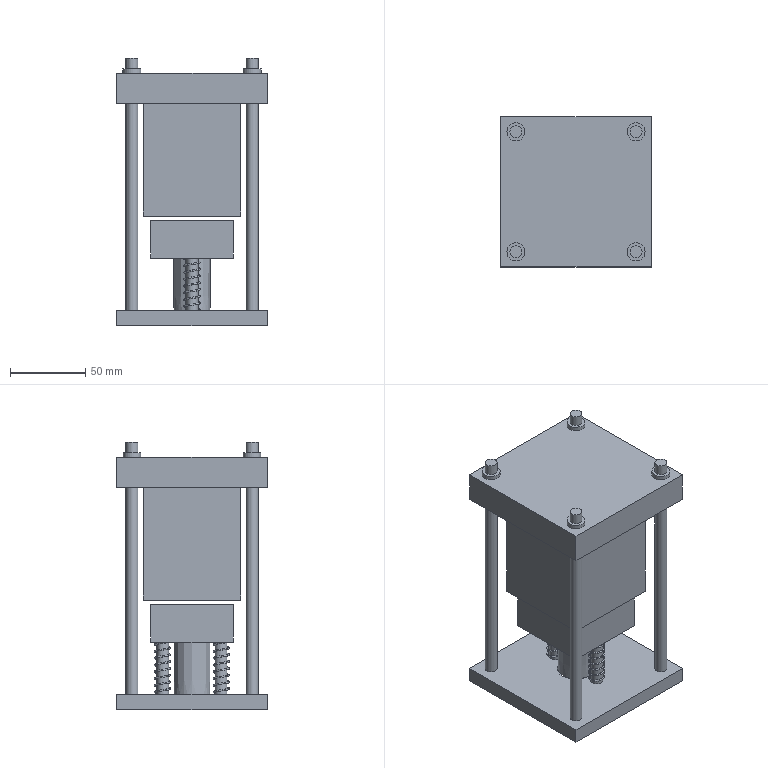Assembly | NX | mm | 6 component files | 10 solids | 363 faces | box 100 x 100 x 178 mm | volume 672900 mm3 | torus 240 | plane 67 | cylinder 49 | cone 7 | commonest cylinder face diameters 8 x22 10 x6 12 x6 20 x4 25.025 x3 35 x2 3 x2 3.5 x2
Bill of materials:
unnamed part 1 | 1 |  | Rectangular block with a square cross-section, taller than it is wide, with a large central through-bore and four small holes in the top face, one near each corner around the bore.
unnamed part 2 | 1 |  | Flat square block with a central through-hole and two helical coil springs sticking out from its bottom face.
unnamed part 3 | 1 |  | Square plate with four long round rods passing through it near the corners, plus several short round pins sticking out from its bottom face.
unnamed part 4 | 1 |  | Square base plate with four corner through-holes, an upright hollow cylindrical tube in the center, and two thin solid rods standing on opposite sides of the tube.
unnamed part 5 | 1 |  | Flanged cylindrical bushing (sleeve with a wider rim at one end) with a central through-bore that has two small notches directly opposite each other.
unnamed part 6 | 1 |  | Stepped cylindrical pin: a larger-diameter lower section with two opposite lengthwise grooves on its outside, a smaller-diameter upper shaft, and a helical coil spring around the upper shaft resting near the shoulder.
Mates:
1. fix | die1 1 component
2. fit | blankdie 1 edge | pads 1 face
3. concentric | blankdie 1 edge | blankdief 1 edge
4. distance | punch 1 face | bolster 1 face
5. concentric | punch 1 edge | bolster 1 edge
6. distance | blankdief 1 face | bolster 1 face
7. parallel | blankdief 1 face | pads 1 face
8. parallel | blankdief 1 face | bolster 1 face
9. parallel | bolster 1 face | die1 1 face